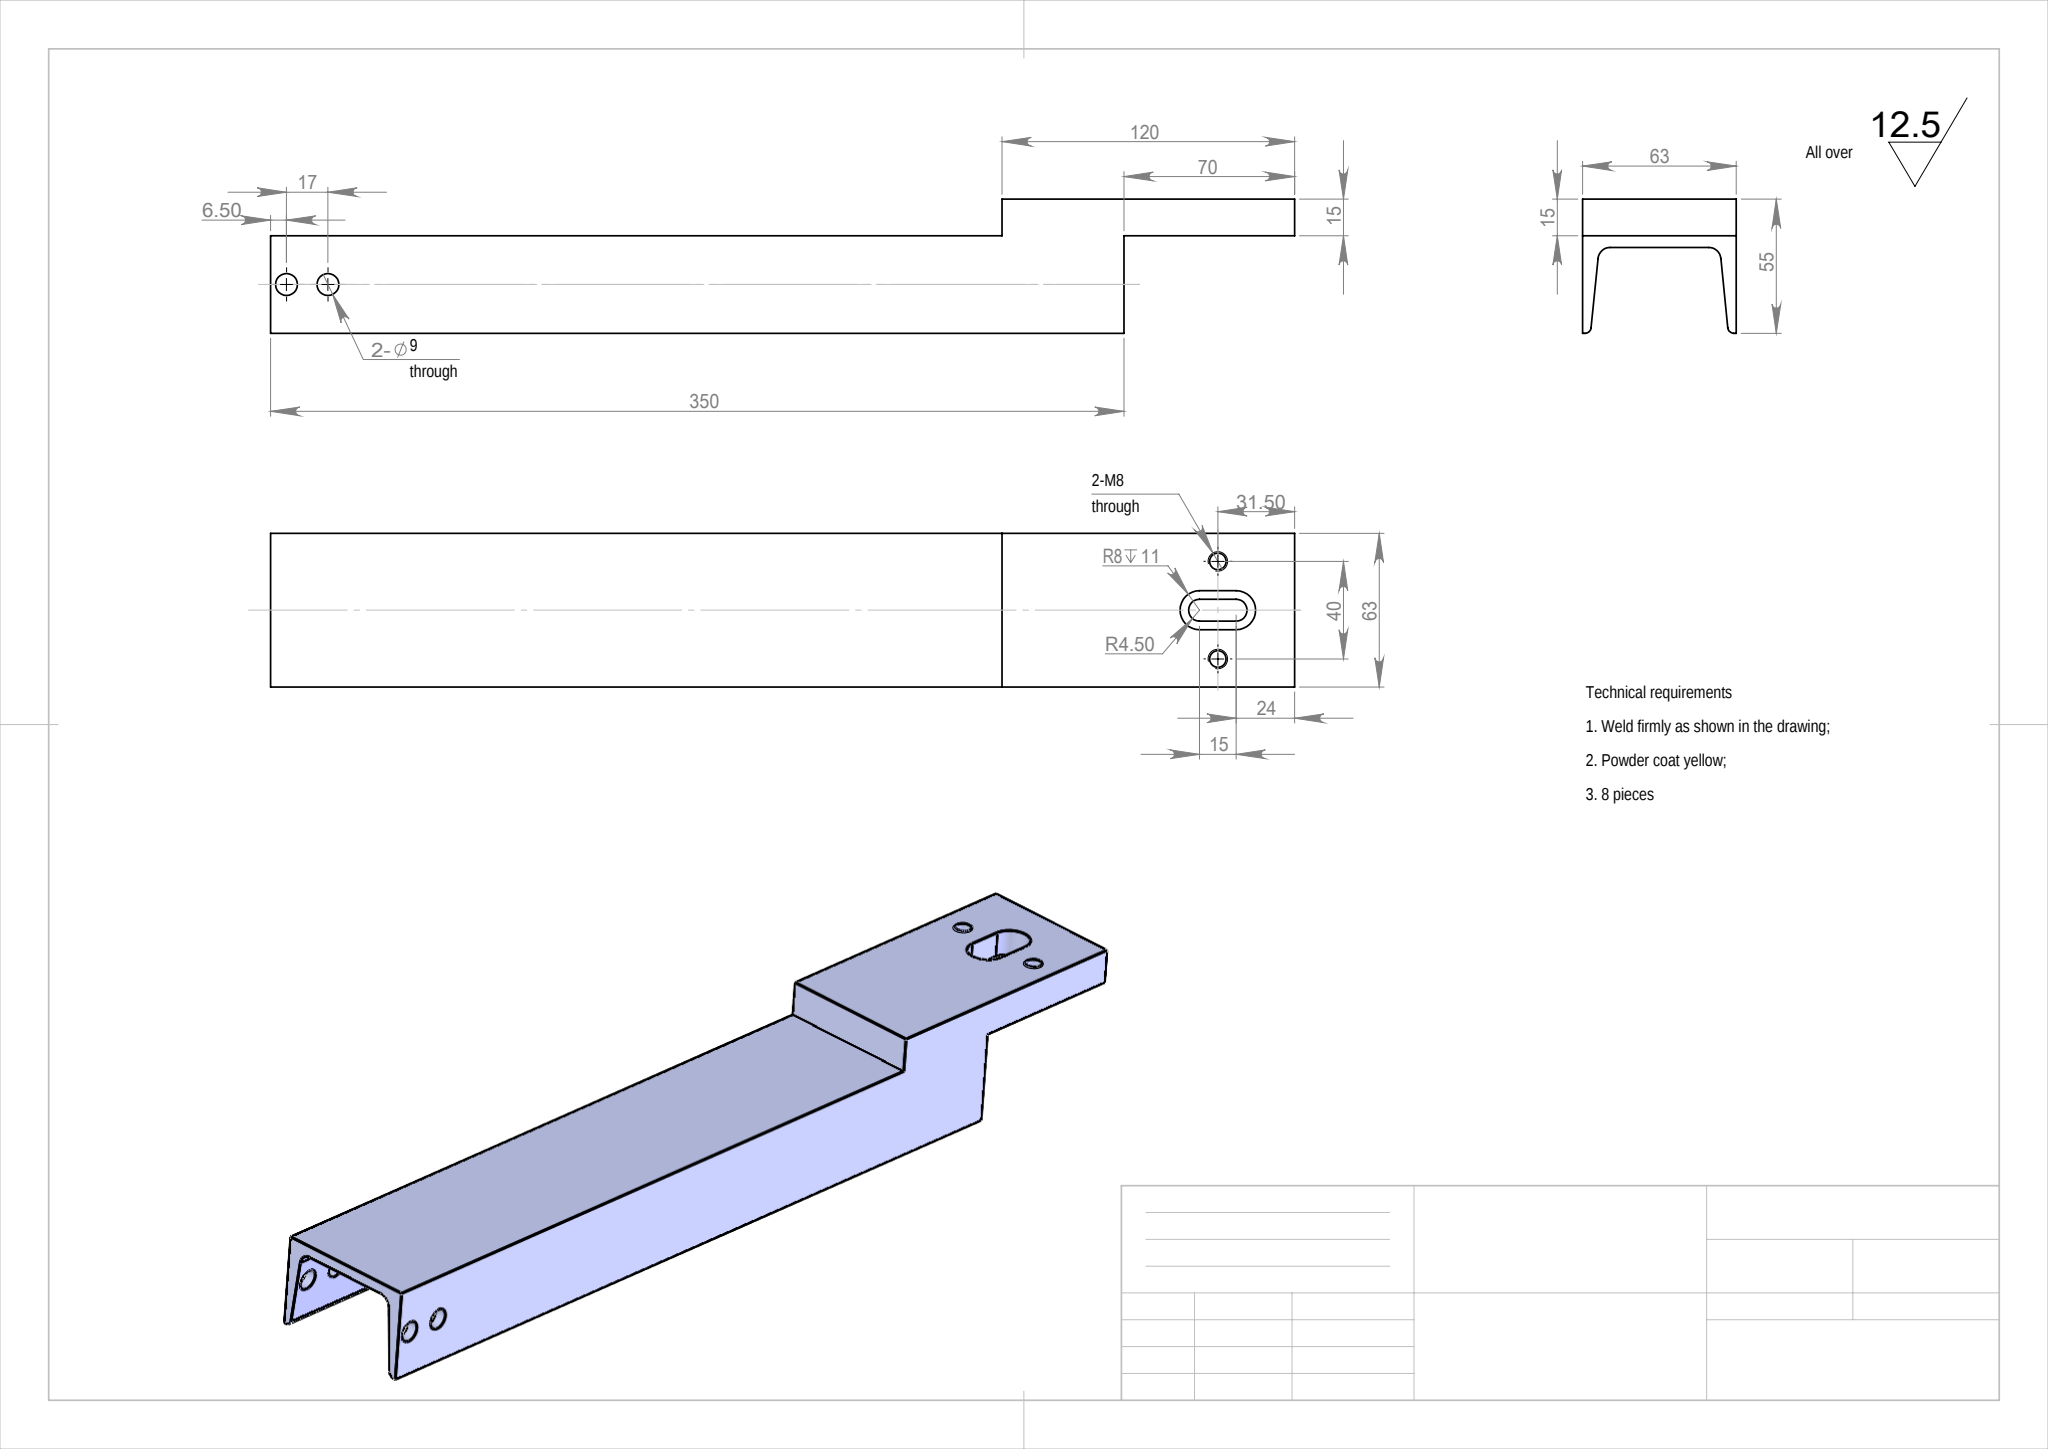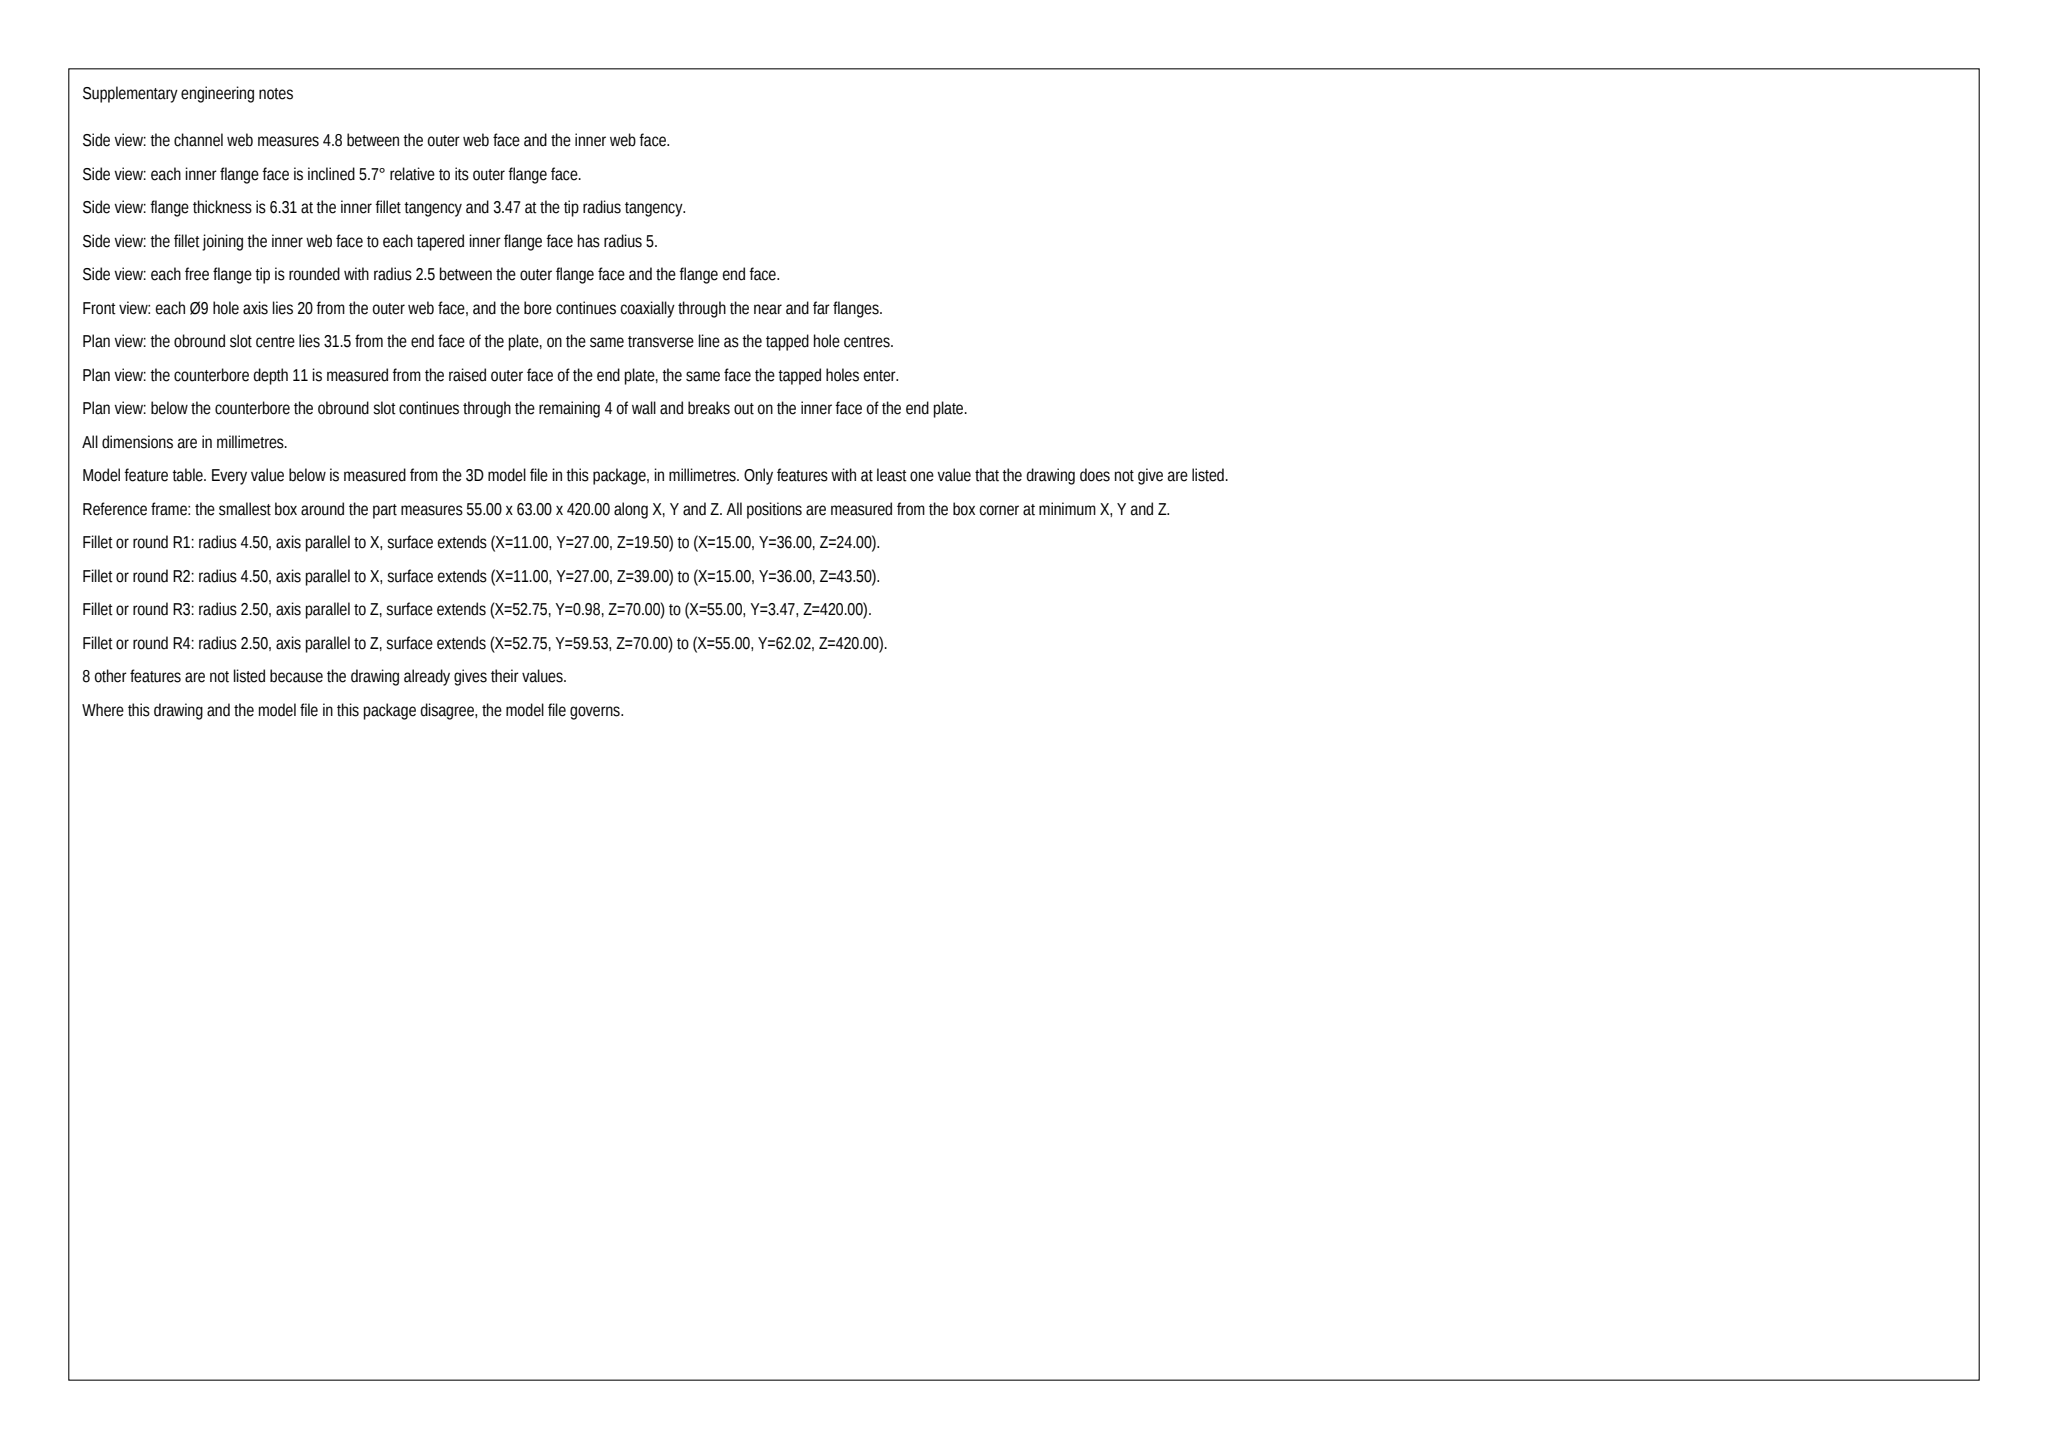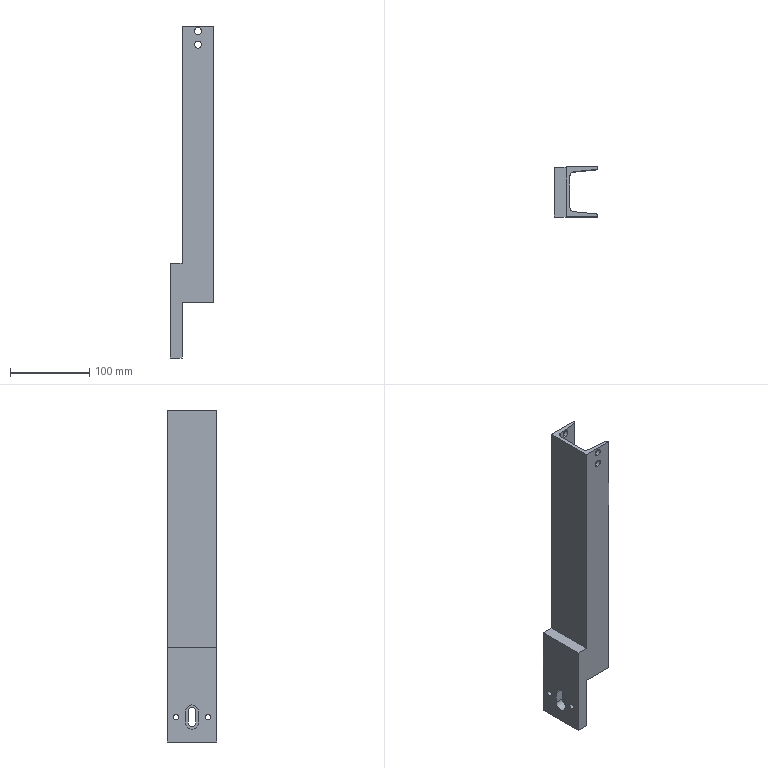Part | SolidWorks | mm | 1 solid | 41 faces | box 55 x 63 x 420 mm | volume 336595 mm3 | cylinder 22 | plane 19 | commonest cylinder face diameters 9 x11 6.8 x4 16 x3 5 x2 10 x2